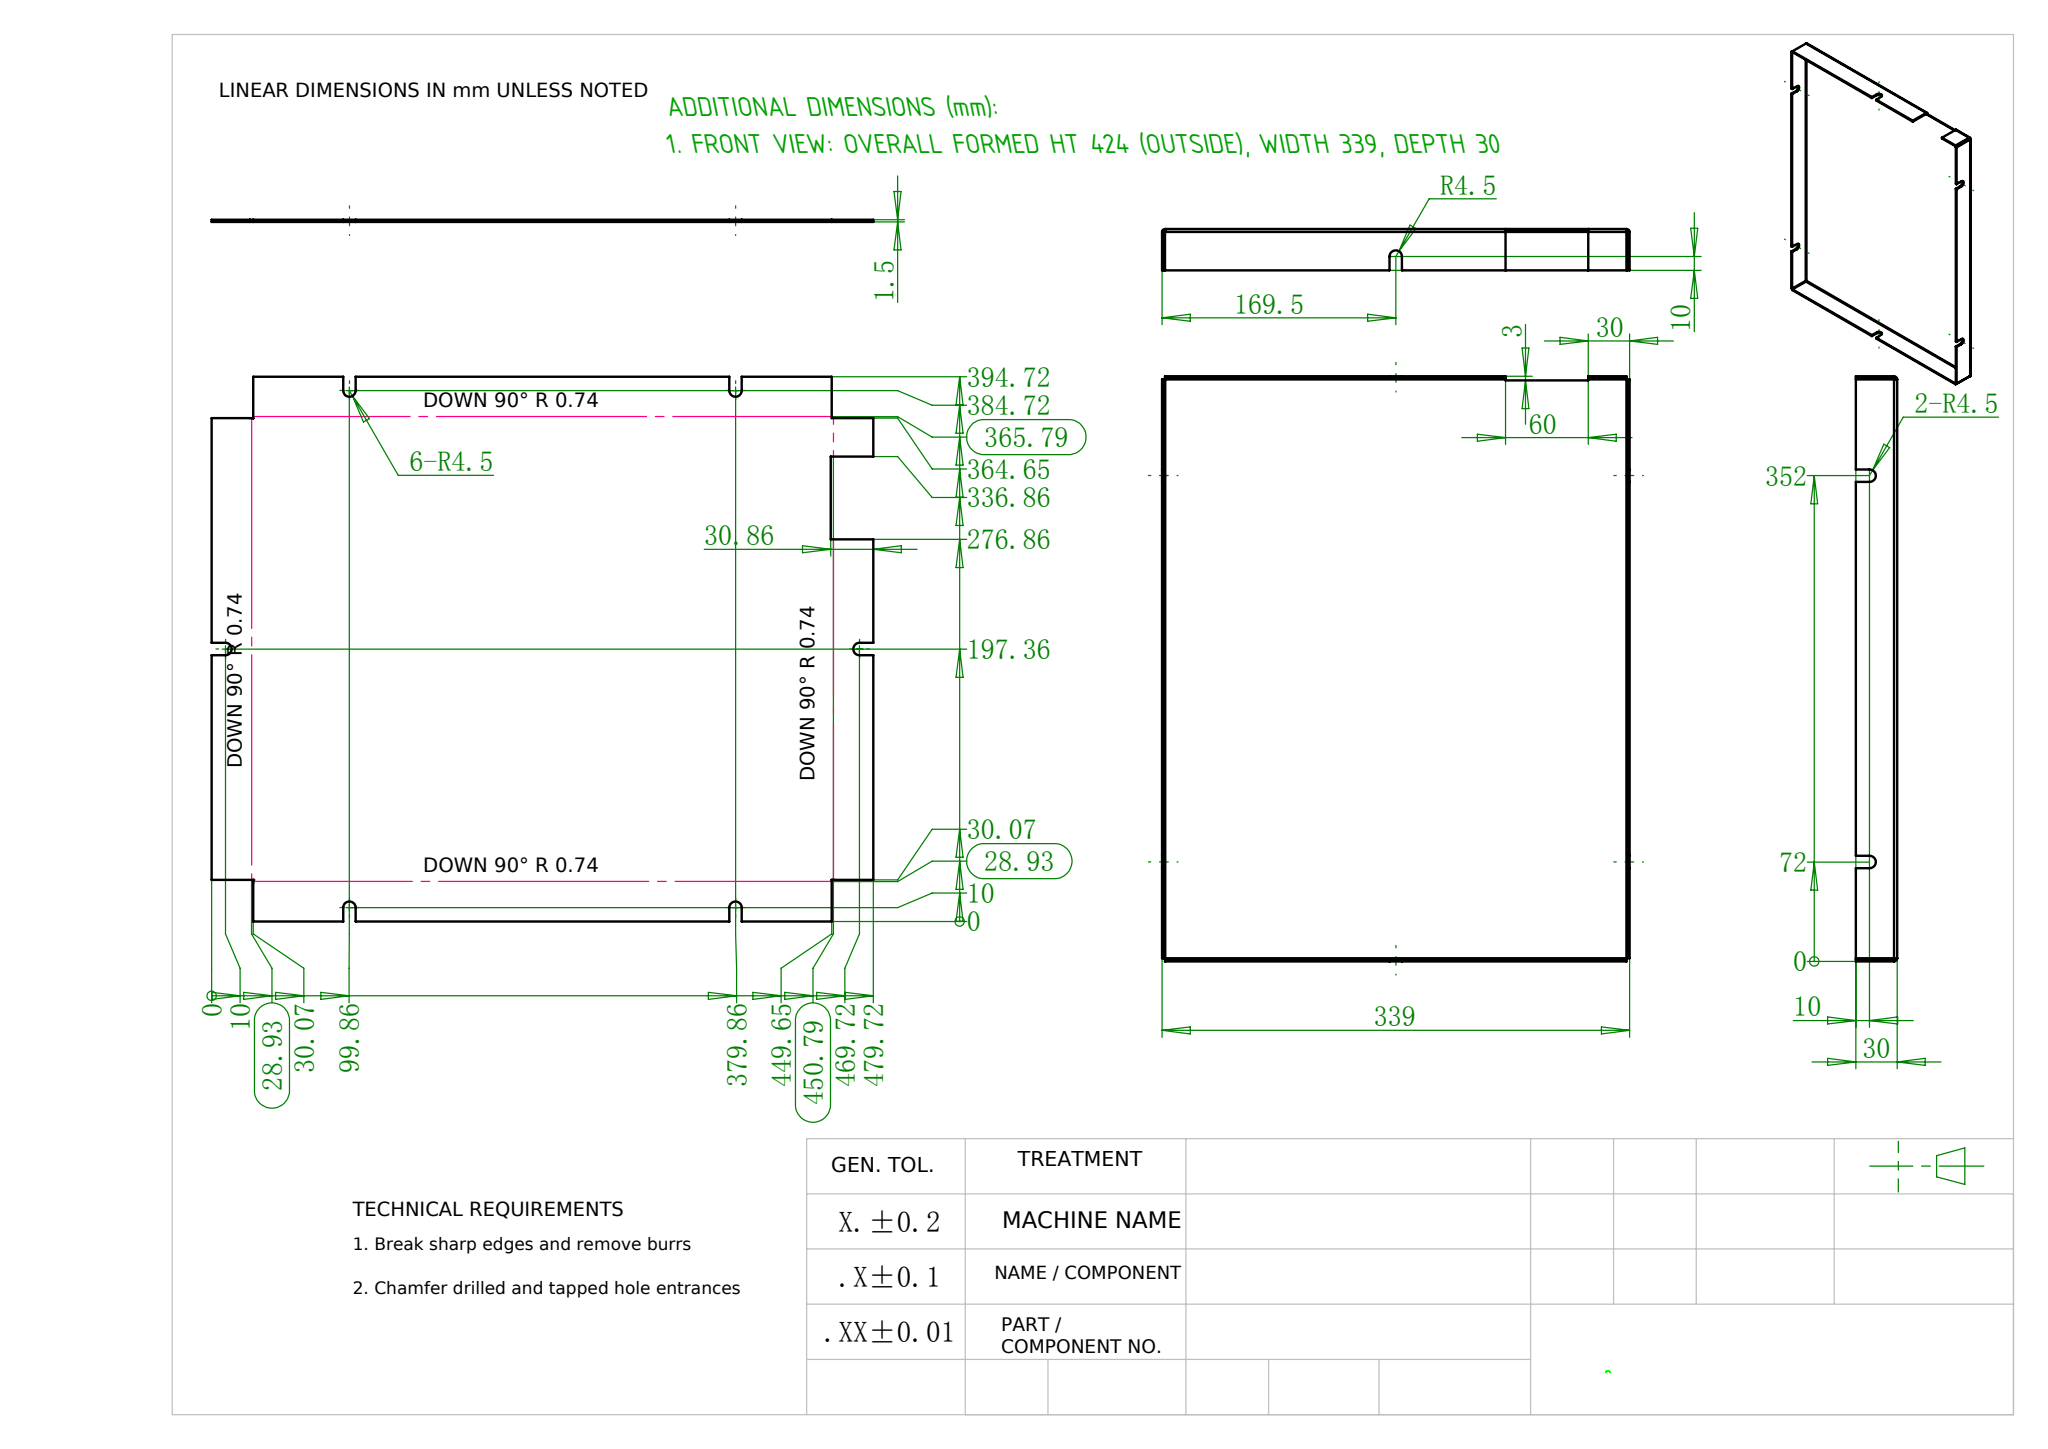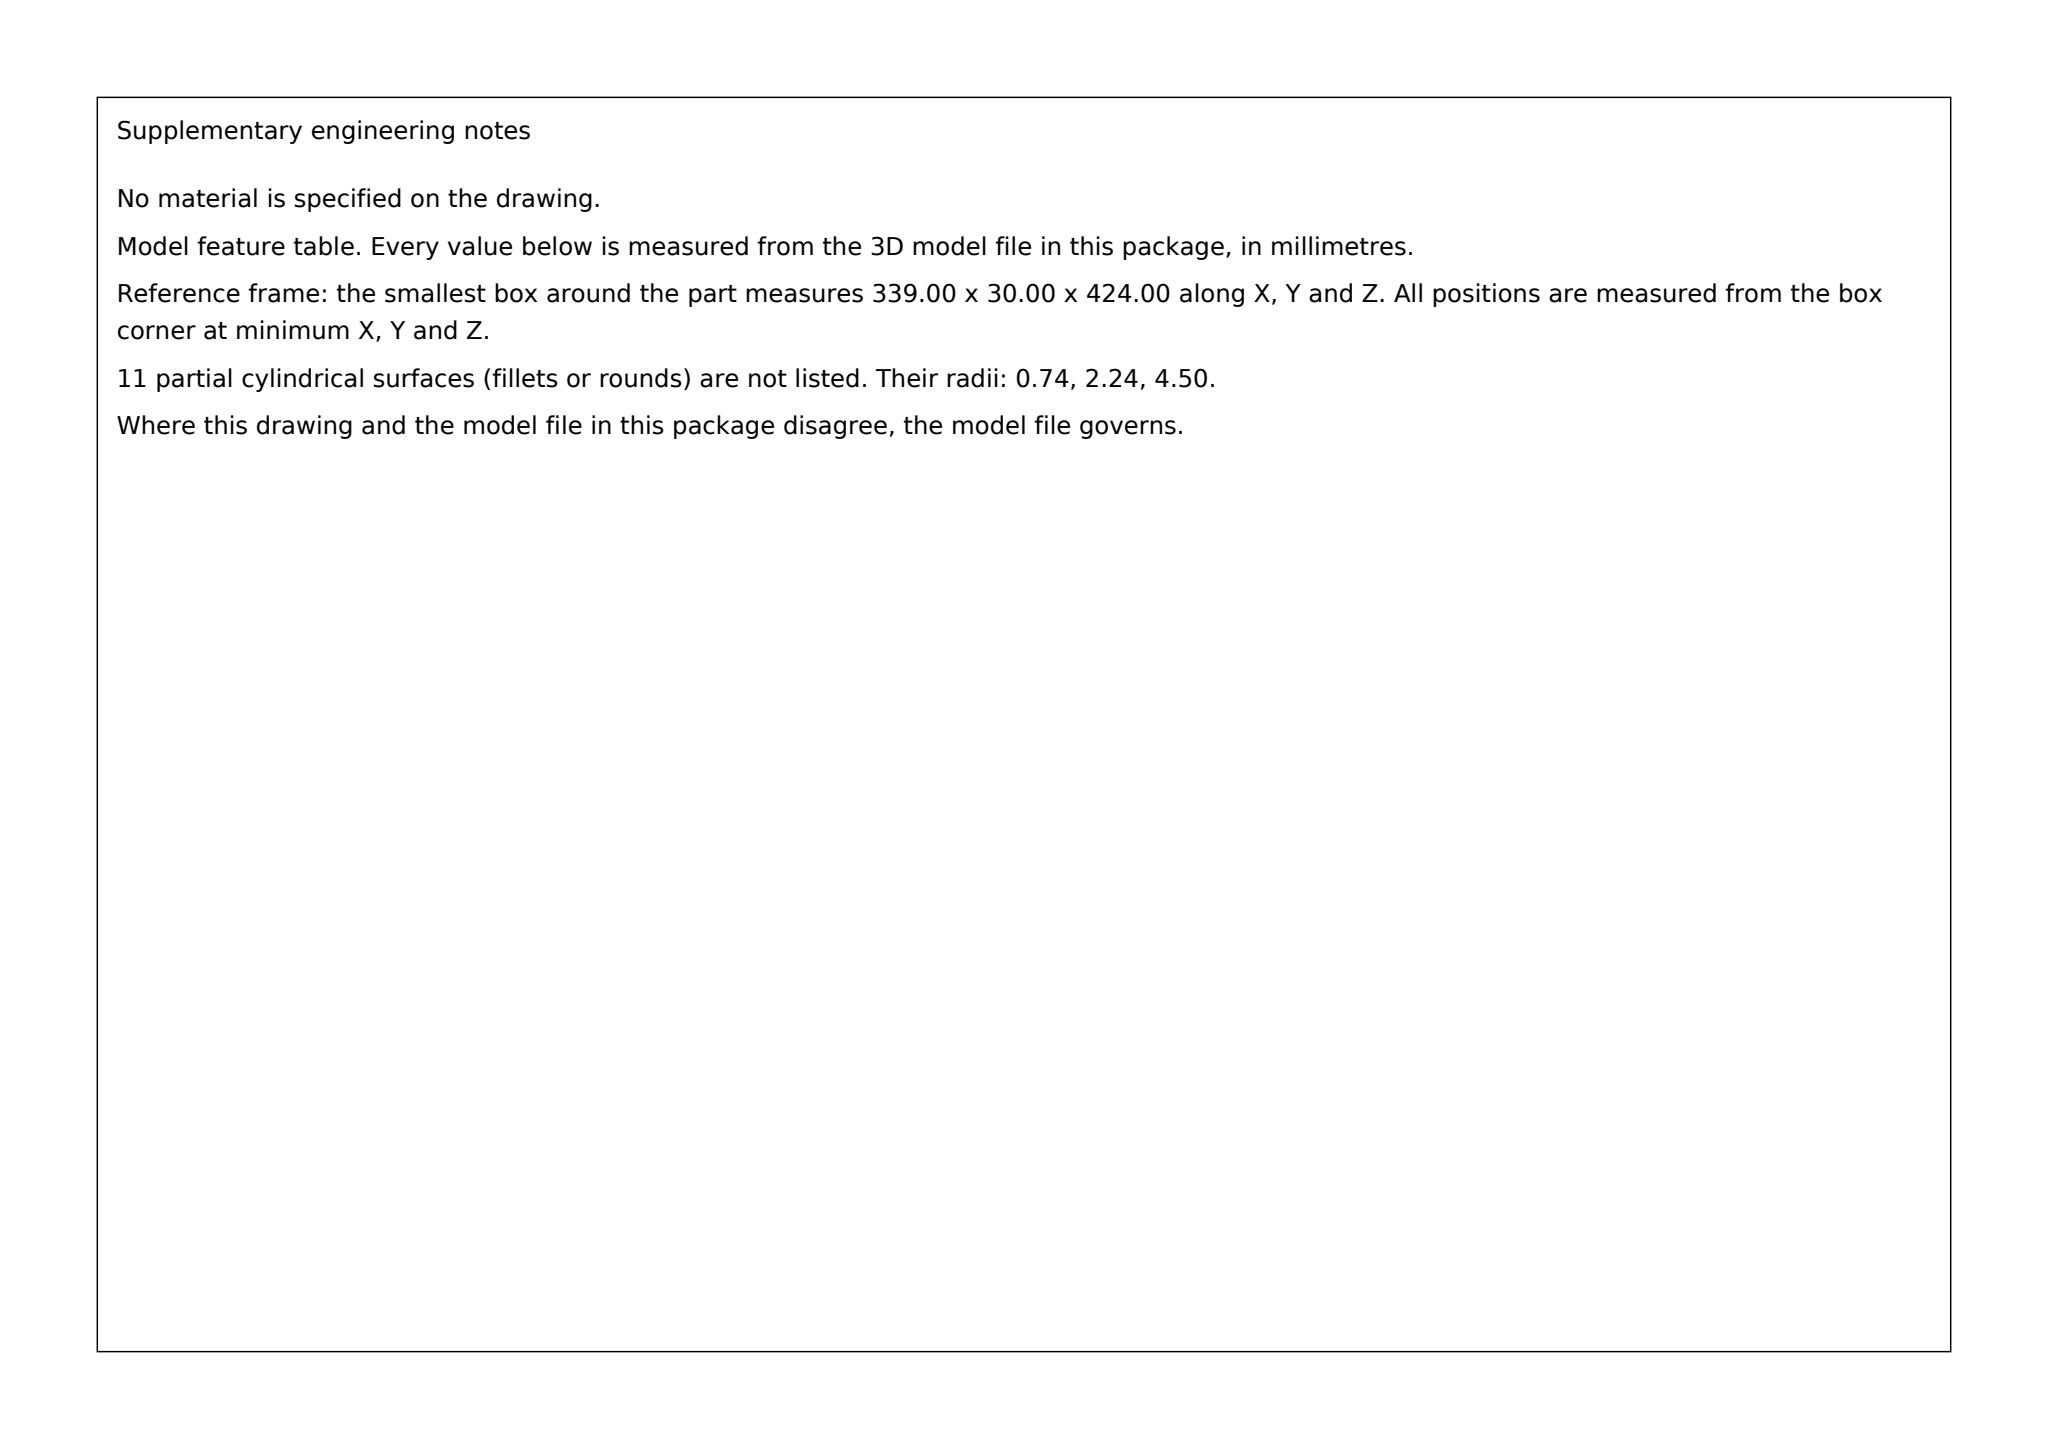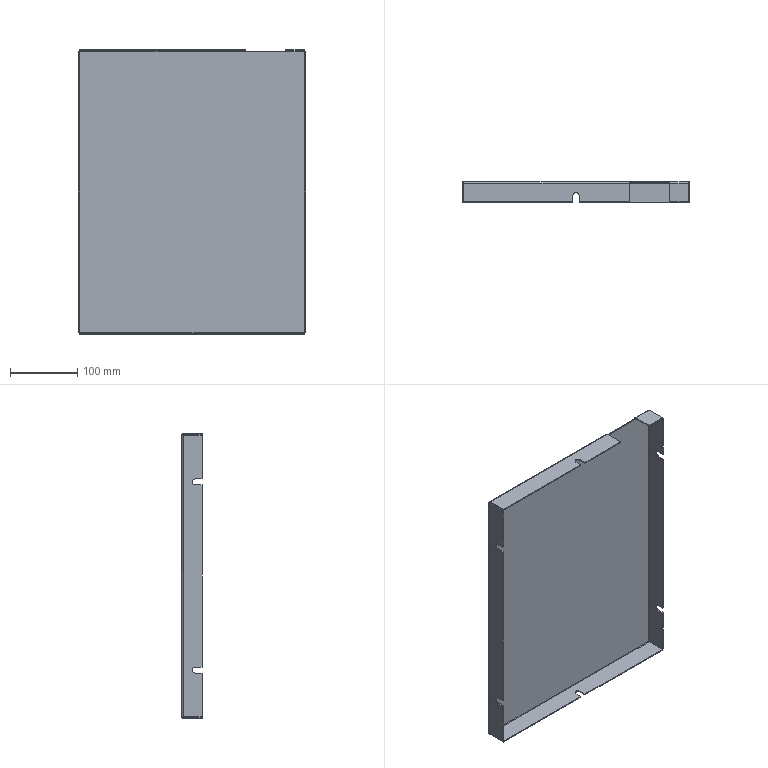Part | SolidWorks | mm | 1 solid | 74 faces | box 339 x 30 x 424 mm | volume 274739 mm3 | plane 50 | cylinder 16 | spline 8 | commonest cylinder face diameters 9 x6 4.473 x5 1.473 x5